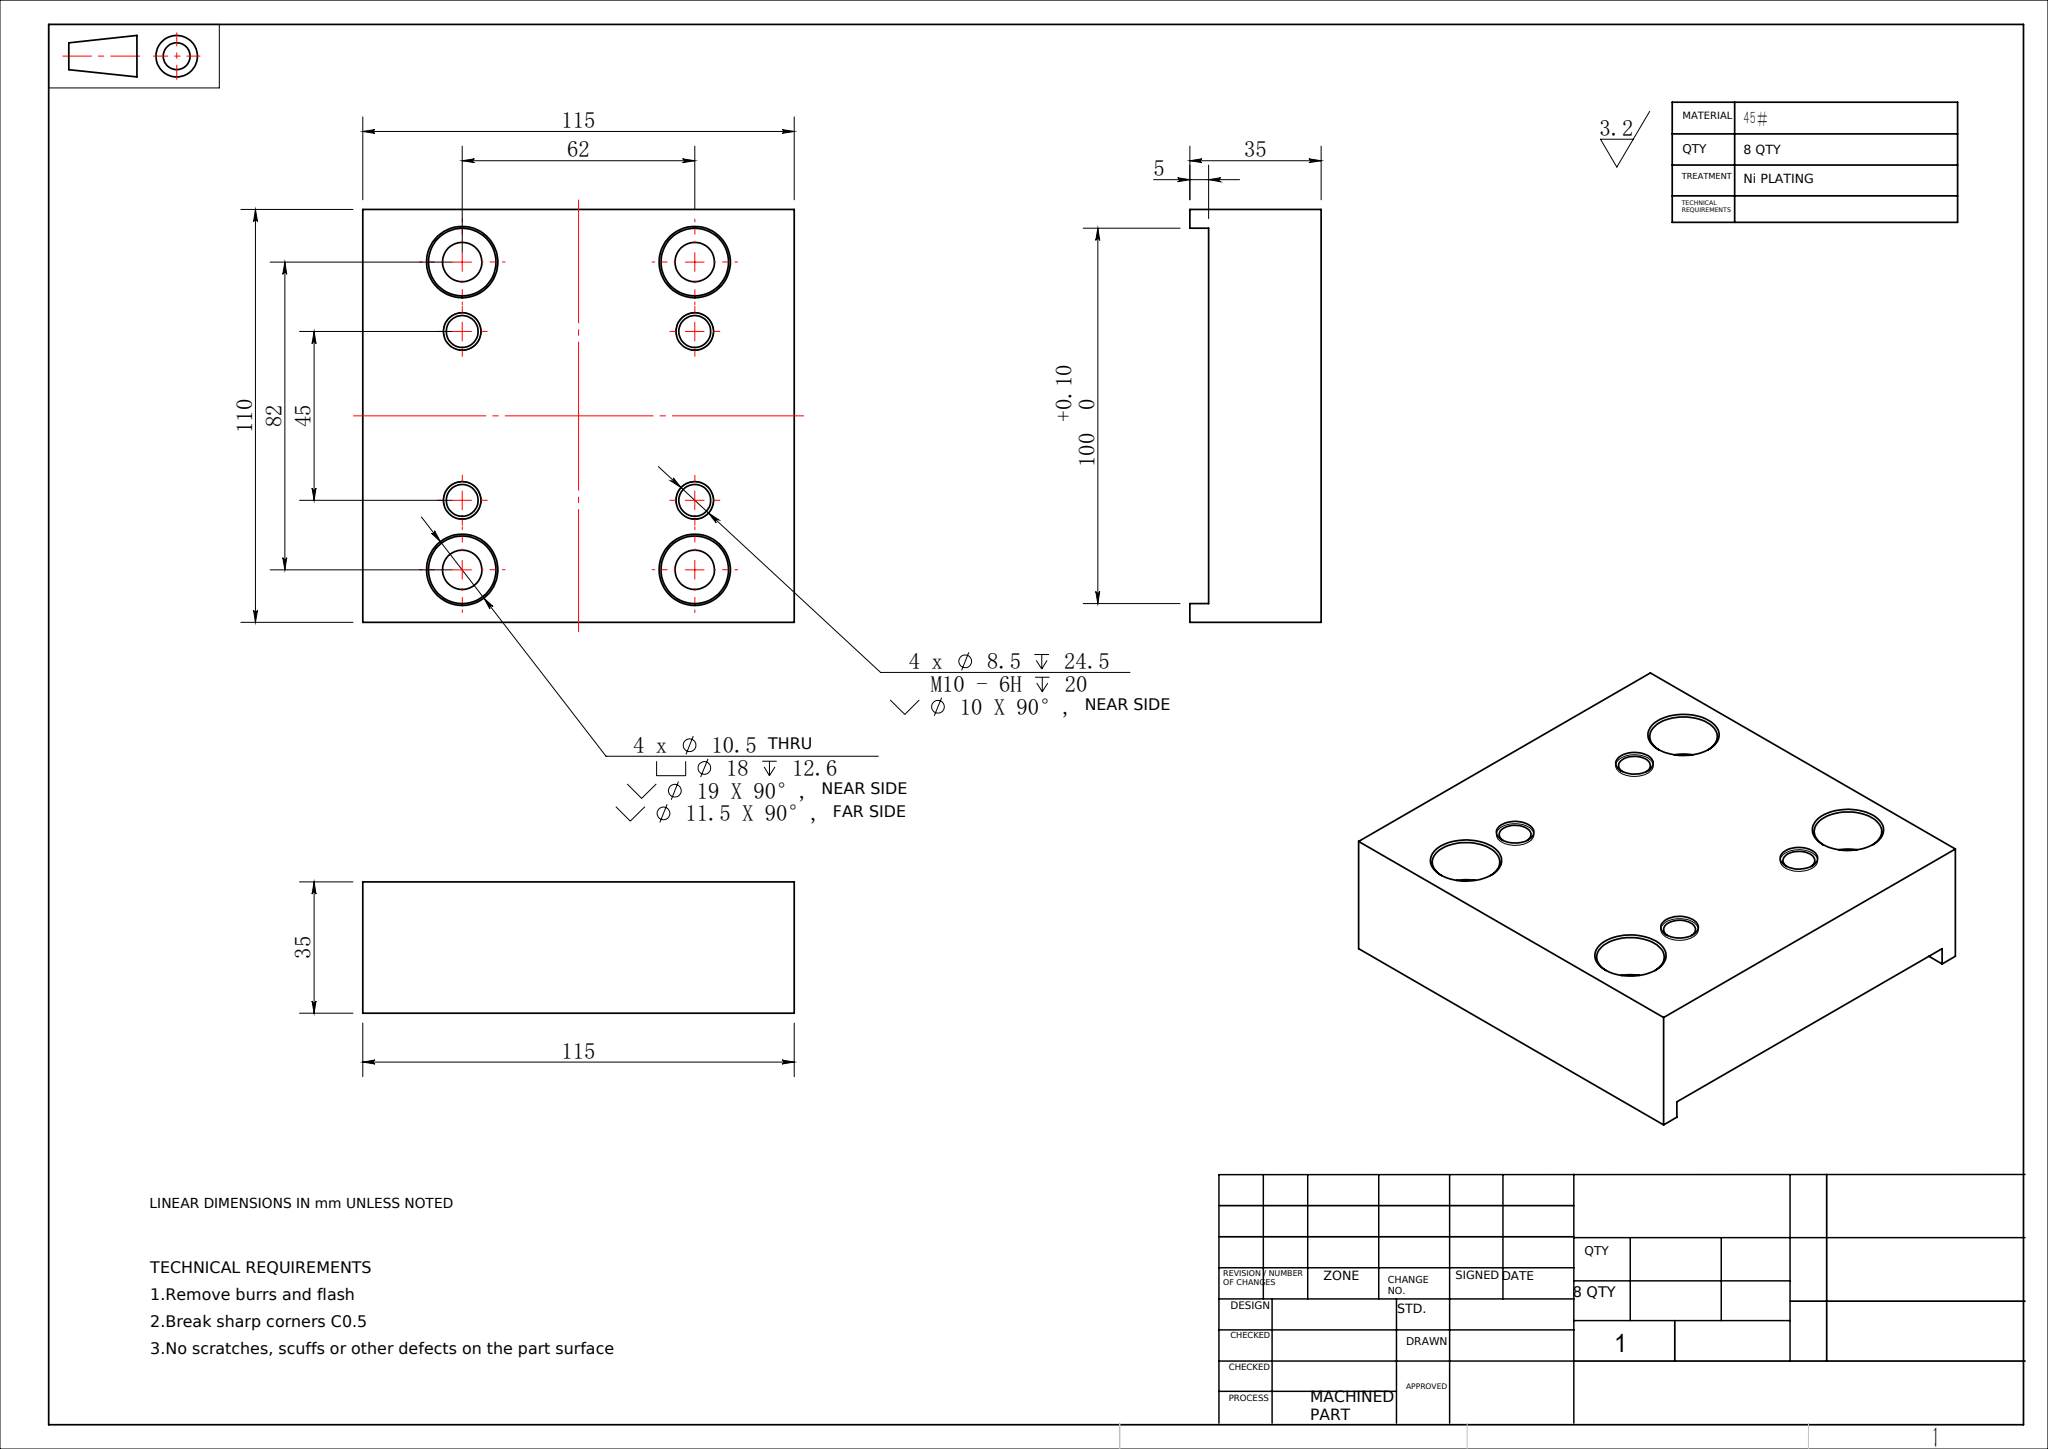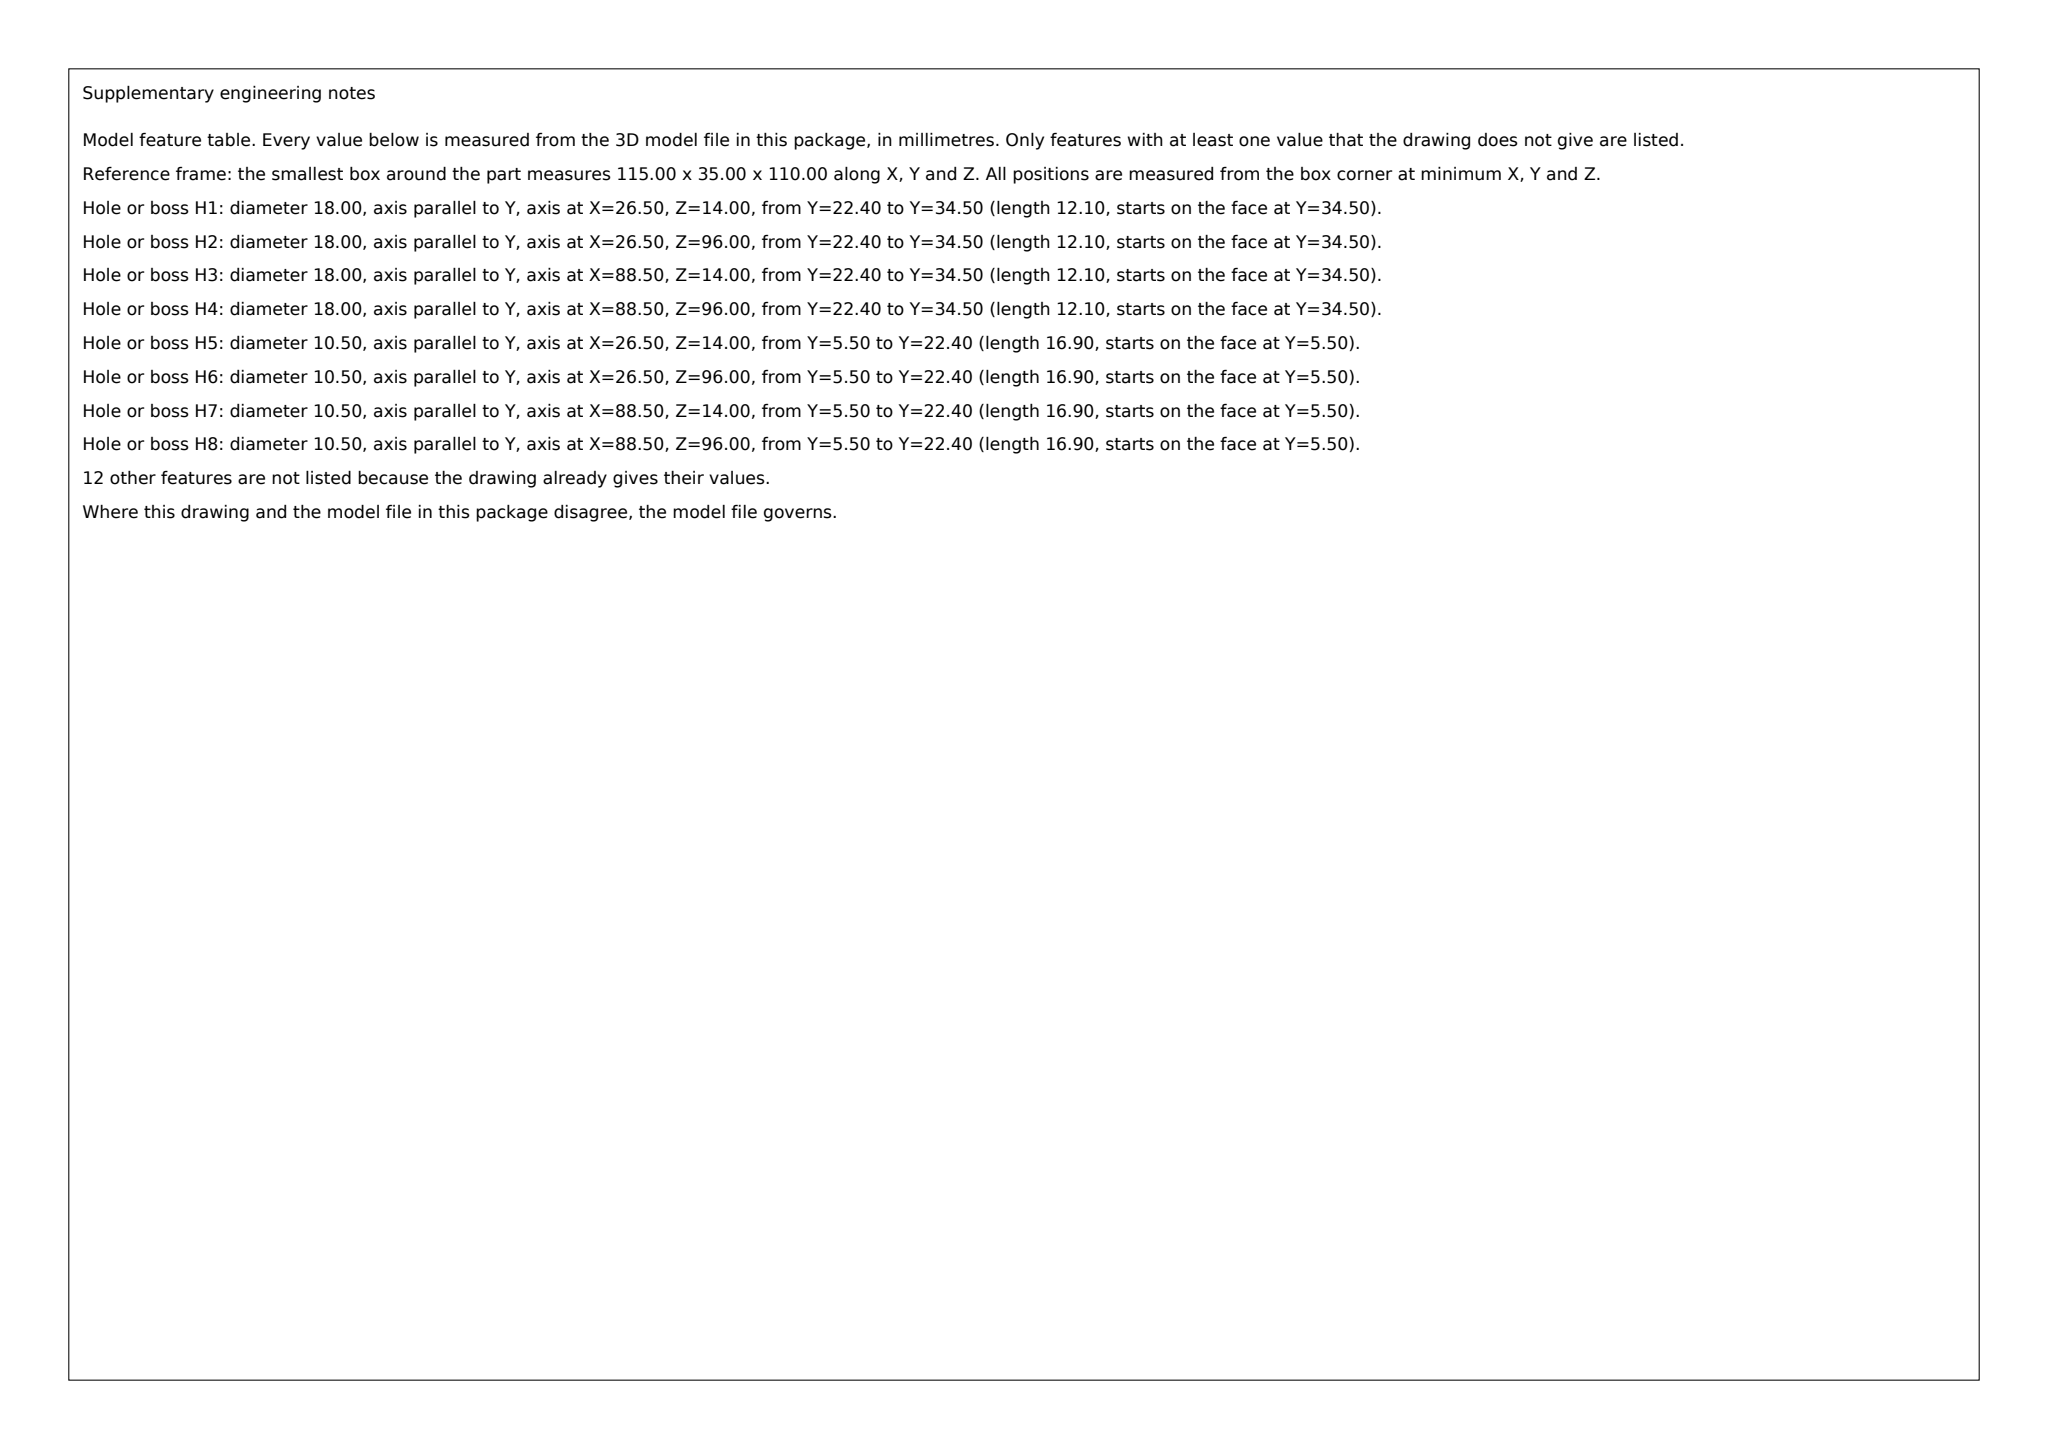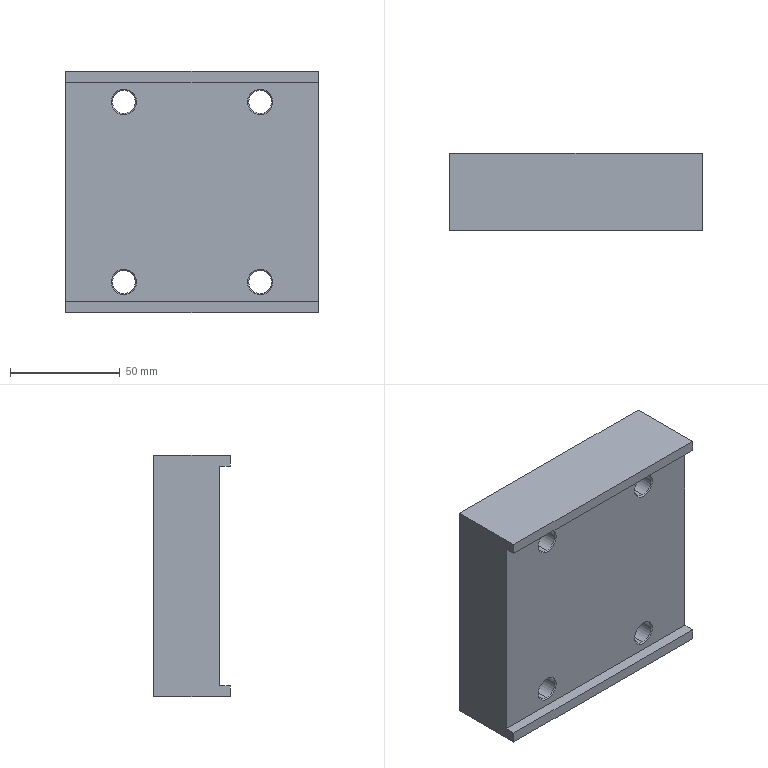Part | SolidWorks | mm | 1 solid | 70 faces | box 115 x 35 x 110 mm | volume 360566 mm3 | cone 32 | cylinder 24 | plane 14 | commonest cylinder face diameters 8.5 x8 18 x8 10.5 x8
build123d program:
from build123d import *

# Parameters (mm, degrees)
SKETCH1_W                                     = 115
SKETCH1_H                                     = 110
BOSS_EXTRUDE1_DEPTH                           = 35
SKETCH2_W                                     = 100
SKETCH2_H                                     = 5
CUT_EXTRUDE1_DEPTH                            = 133.193
M10_HEX_SOCKET_HEAD_CAP_SCREW_CBORE1_AT_COUNT = 2
M10_HEX_SOCKET_HEAD_CAP_SCREW_CBORE1_AT_PITCH = 62
M10_HEX_SOCKET_HEAD_CAP_SCREW_CBORE1_2_COUNT  = 2
M10_HEX_SOCKET_HEAD_CAP_SCREW_CBORE1_2_PITCH  = 102.801
M10_HEX_SOCKET_HEAD_CAP_SCREW_CBORE1_3_COUNT  = 2
M10_HEX_SOCKET_HEAD_CAP_SCREW_CBORE1_3_PITCH  = 82
M10_TAPPED_HOLE1_D                            = 8.5
M10_TAPPED_HOLE1_DEPTH                        = 24.5
M10_TAPPED_HOLE1_CSINK_D                      = 10
M10_TAPPED_HOLE1_CSINK_ANGLE                  = 90
M10_TAPPED_HOLE1_TIP                          = 2.554


with BuildPart() as part:
    # Sketch1 → Boss-Extrude1 (new body)
    with BuildSketch(Plane(origin=(0, 0, 0), x_dir=(1, 0, 0), z_dir=(0, 1, 0))):
        Rectangle(SKETCH1_W, SKETCH1_H)
    extrude(amount=BOSS_EXTRUDE1_DEPTH)

    # Sketch2 → Cut-Extrude1 (cut, through all)
    with BuildSketch(Plane(origin=(57.5, 0, 0), x_dir=(0, 0, -1), z_dir=(1, 0, 0))):
        with Locations((0, 2.5)):
            Rectangle(SKETCH2_W, SKETCH2_H)
    extrude(amount=-CUT_EXTRUDE1_DEPTH, mode=Mode.SUBTRACT)

    # Sketch4 → M10 Hex Socket Head Cap Screw CBORE1 (revolve, cut)
    with BuildSketch(Plane(origin=(31, 35, -41), x_dir=(0, 0, 1), z_dir=(1, 0, 0))):
        Polygon((0, 0), (0, 30), (5.75, 30), (5.25, 29.5), (5.25, 12.6), (9, 12.6), (9, 0.5), (9.5, 0), align=None)
    m10_hex_socket_head_cap_screw_cbore1 = revolve(axis=Axis((31, 41.35, -41), (0, -1, 0)), mode=Mode.SUBTRACT)

    # M10 Hex Socket Head Cap Screw CBORE1 at: M10 Hex Socket Head Cap Screw CBORE1 ×2
    with Locations(*[(-i * M10_HEX_SOCKET_HEAD_CAP_SCREW_CBORE1_AT_PITCH, 0, 0) for i in range(1, M10_HEX_SOCKET_HEAD_CAP_SCREW_CBORE1_AT_COUNT)]):
        add(m10_hex_socket_head_cap_screw_cbore1, mode=Mode.SUBTRACT)

    # M10 Hex Socket Head Cap Screw CBORE1 2: M10 Hex Socket Head Cap Screw CBORE1 ×2
    with Locations(*[Vector(-0.6031, 0, 0.7977) * (i * M10_HEX_SOCKET_HEAD_CAP_SCREW_CBORE1_2_PITCH) for i in range(1, M10_HEX_SOCKET_HEAD_CAP_SCREW_CBORE1_2_COUNT)]):
        add(m10_hex_socket_head_cap_screw_cbore1, mode=Mode.SUBTRACT)

    # M10 Hex Socket Head Cap Screw CBORE1 3: M10 Hex Socket Head Cap Screw CBORE1 ×2
    with Locations(*[(0, 0, i * M10_HEX_SOCKET_HEAD_CAP_SCREW_CBORE1_3_PITCH) for i in range(1, M10_HEX_SOCKET_HEAD_CAP_SCREW_CBORE1_3_COUNT)]):
        add(m10_hex_socket_head_cap_screw_cbore1, mode=Mode.SUBTRACT)

    # M10 Tapped Hole1
    with Locations(Plane(origin=(0, 35, 0), x_dir=(1, 0, 0), z_dir=(0, 1, 0))):
        with Locations((-31, 22.5), (31, 22.5), (31, -22.5), (-31, -22.5)):
            CounterSinkHole(M10_TAPPED_HOLE1_D / 2, M10_TAPPED_HOLE1_CSINK_D / 2, depth=M10_TAPPED_HOLE1_DEPTH, counter_sink_angle=M10_TAPPED_HOLE1_CSINK_ANGLE)
            with Locations((0, 0, -(M10_TAPPED_HOLE1_DEPTH + M10_TAPPED_HOLE1_TIP / 2))):  # 118° drill point
                Cone(0, M10_TAPPED_HOLE1_D / 2, M10_TAPPED_HOLE1_TIP, mode=Mode.SUBTRACT)


solid = part.part